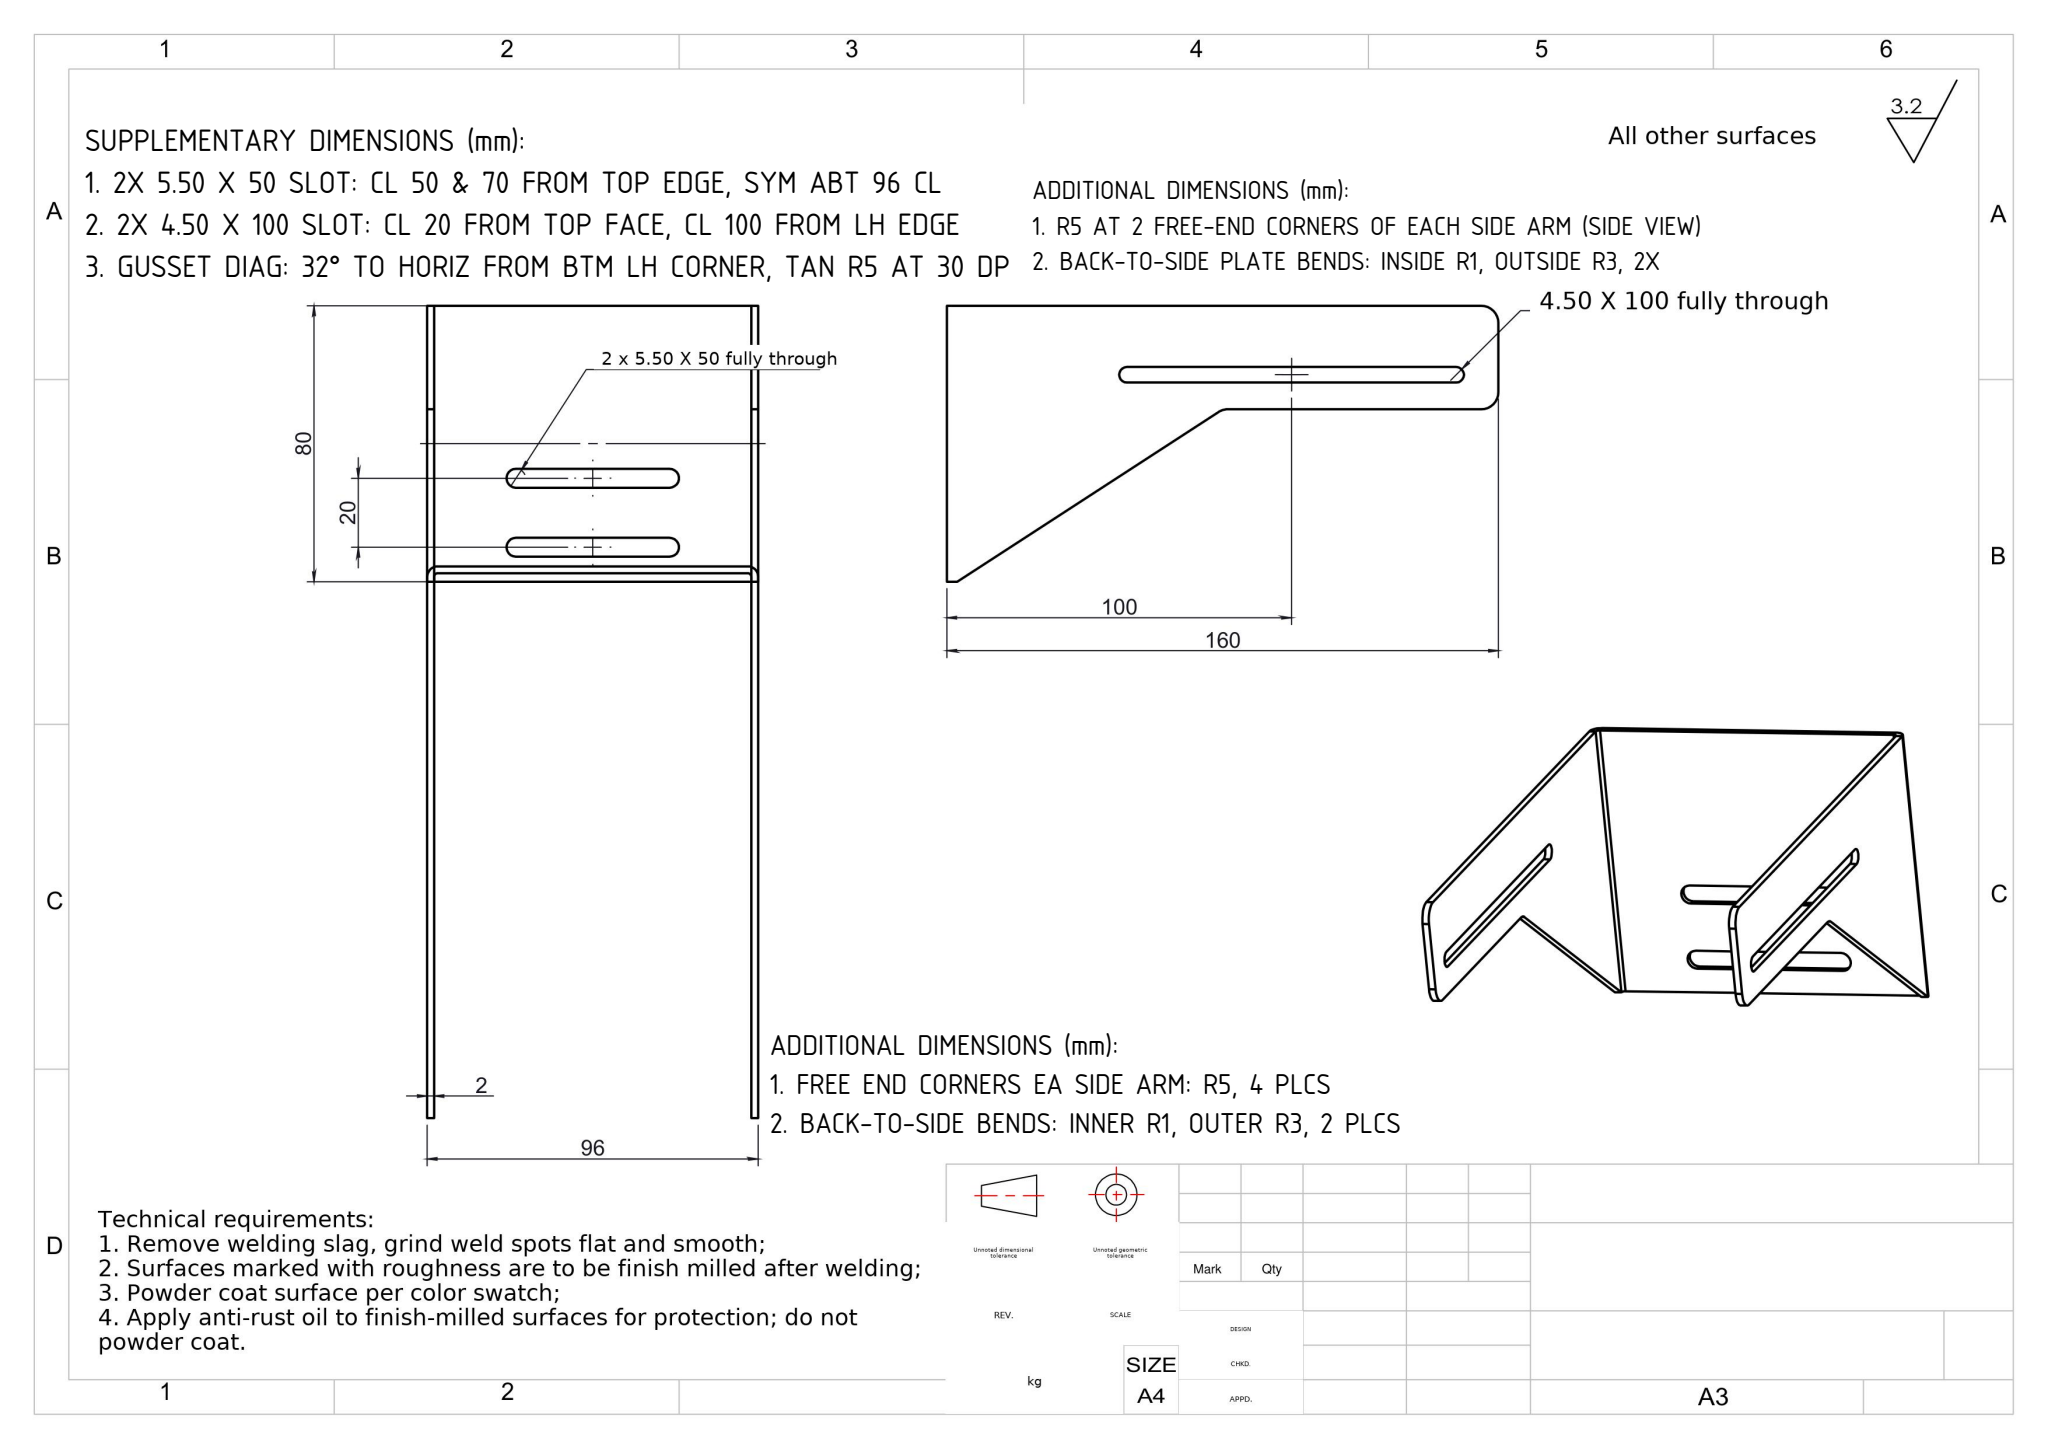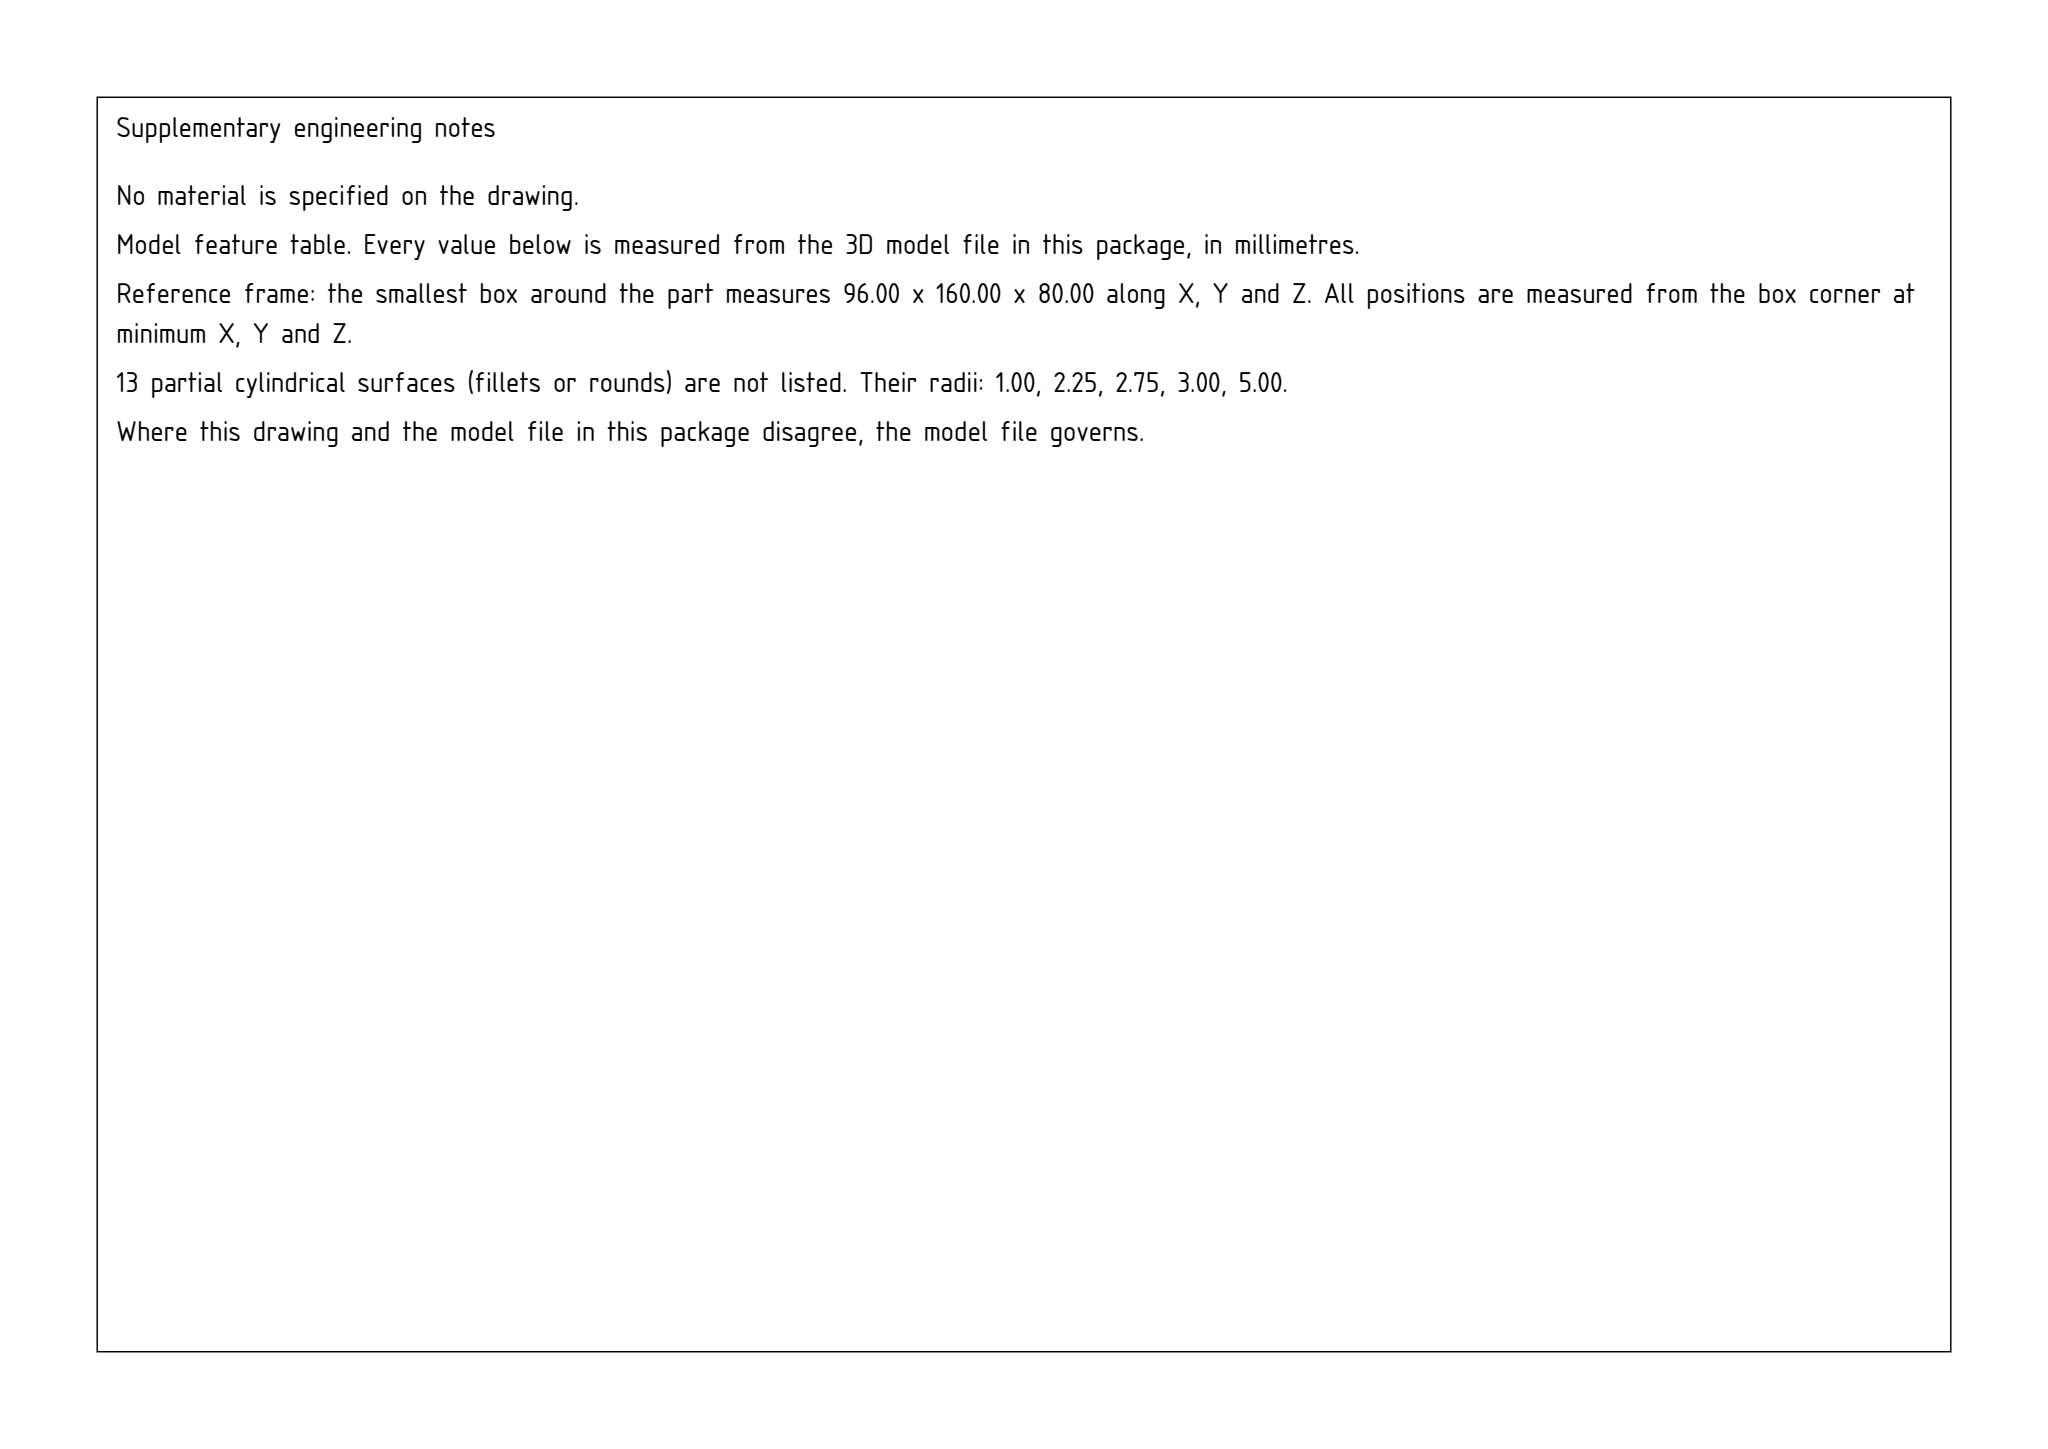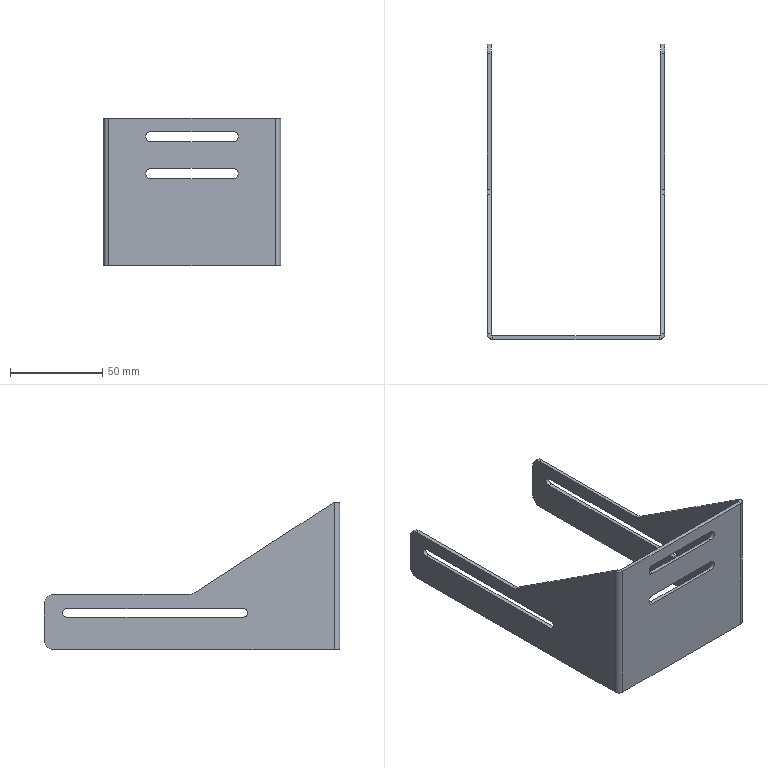Part | SolidWorks | mm | 1 solid | 46 faces | box 96 x 160 x 80 mm | volume 39047 mm3 | plane 28 | cylinder 18 | commonest cylinder face diameters 10 x6 5.5 x4 4.5 x4 6 x2 2 x2